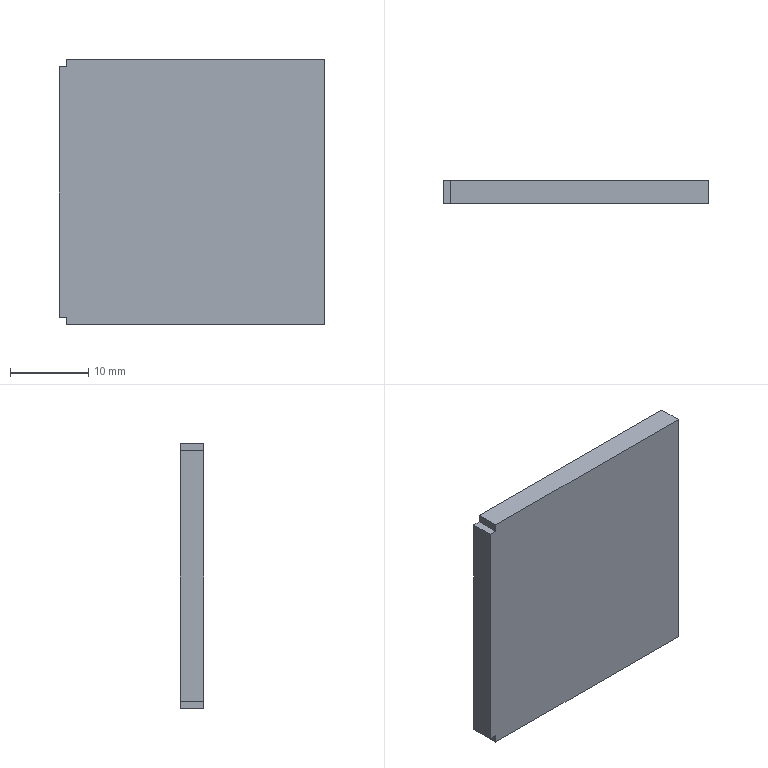Component | SolidWorks | CCQ-1.1-8WeldedPlate-4 | 1 solid | 10 faces | box 34 x 3 x 34 mm | volume 3462 mm3 | plane 10 | material 304
STEP:
#1=COLOUR_RGB('',0.7922,0.8196,0.9333);
#2=FILL_AREA_STYLE_COLOUR('',#1);
#3=FILL_AREA_STYLE('',(#2));
#4=SURFACE_STYLE_FILL_AREA(#3);
#5=SURFACE_SIDE_STYLE('',(#4));
#6=SURFACE_STYLE_USAGE(.BOTH.,#5);
#7=PRESENTATION_STYLE_ASSIGNMENT((#6));
#8=CARTESIAN_POINT('',(-25.866,-21.28,0.6299));
#9=VERTEX_POINT('',#8);
#10=CARTESIAN_POINT('',(-25.866,-21.398,0.6299));
#11=VERTEX_POINT('',#10);
#12=CARTESIAN_POINT('',(-25.866,-21.28,0.6299));
#13=DIRECTION('',(0.,-1.,0.));
#14=VECTOR('',#13,39.37);
#15=LINE('',#12,#14);
#16=EDGE_CURVE('',#9,#11,#15,.T.);
#17=ORIENTED_EDGE('',*,*,#16,.F.);
#18=CARTESIAN_POINT('',(-25.866,-21.28,-0.6299));
#19=VERTEX_POINT('',#18);
#20=CARTESIAN_POINT('',(-25.866,-21.28,-0.6693));
#21=DIRECTION('',(0.,-0.,-1.));
#22=VECTOR('',#21,39.37);
#23=LINE('',#20,#22);
#24=EDGE_CURVE('',#9,#19,#23,.T.);
#25=ORIENTED_EDGE('',*,*,#24,.T.);
#26=CARTESIAN_POINT('',(-25.866,-21.398,-0.6299));
#27=VERTEX_POINT('',#26);
#28=CARTESIAN_POINT('',(-25.866,-21.28,-0.6299));
#29=DIRECTION('',(-0.,1.,-0.));
#30=VECTOR('',#29,39.37);
#31=LINE('',#28,#30);
#32=EDGE_CURVE('',#27,#19,#31,.T.);
#33=ORIENTED_EDGE('',*,*,#32,.F.);
#34=CARTESIAN_POINT('',(-25.866,-21.398,-0.6693));
#35=DIRECTION('',(0.,-0.,-1.));
#36=VECTOR('',#35,39.37);
#37=LINE('',#34,#36);
#38=EDGE_CURVE('',#11,#27,#37,.T.);
#39=ORIENTED_EDGE('',*,*,#38,.F.);
#40=EDGE_LOOP('',(#17,#25,#33,#39));
#41=FACE_OUTER_BOUND('',#40,.T.);
#42=CARTESIAN_POINT('',(-25.866,-21.28,-0.6693));
#43=DIRECTION('',(-1.,-0.,-0.));
#44=DIRECTION('',(0.,-0.,-1.));
#45=AXIS2_PLACEMENT_3D('',#42,#43,#44);
#46=PLANE('',#45);
#47=ADVANCED_FACE('',(#41),#46,.T.);
#48=CARTESIAN_POINT('',(-25.827,-21.398,0.6693));
#49=VERTEX_POINT('',#48);
#50=CARTESIAN_POINT('',(-25.827,-21.28,0.6693));
#51=VERTEX_POINT('',#50);
#52=CARTESIAN_POINT('',(-25.827,-21.28,0.6693));
#53=DIRECTION('',(-0.,1.,-0.));
#54=VECTOR('',#53,39.37);
#55=LINE('',#52,#54);
#56=EDGE_CURVE('',#49,#51,#55,.T.);
#57=ORIENTED_EDGE('',*,*,#56,.F.);
#58=CARTESIAN_POINT('',(-24.528,-21.398,0.6693));
#59=VERTEX_POINT('',#58);
#60=CARTESIAN_POINT('',(-24.528,-21.398,0.6693));
#61=DIRECTION('',(-1.,-0.,0.));
#62=VECTOR('',#61,39.37);
#63=LINE('',#60,#62);
#64=EDGE_CURVE('',#59,#49,#63,.T.);
#65=ORIENTED_EDGE('',*,*,#64,.F.);
#66=CARTESIAN_POINT('',(-24.528,-21.28,0.6693));
#67=VERTEX_POINT('',#66);
#68=CARTESIAN_POINT('',(-24.528,-21.28,0.6693));
#69=DIRECTION('',(0.,-1.,0.));
#70=VECTOR('',#69,39.37);
#71=LINE('',#68,#70);
#72=EDGE_CURVE('',#67,#59,#71,.T.);
#73=ORIENTED_EDGE('',*,*,#72,.F.);
#74=CARTESIAN_POINT('',(-24.528,-21.28,0.6693));
#75=DIRECTION('',(-1.,-0.,0.));
#76=VECTOR('',#75,39.37);
#77=LINE('',#74,#76);
#78=EDGE_CURVE('',#67,#51,#77,.T.);
#79=ORIENTED_EDGE('',*,*,#78,.T.);
#80=EDGE_LOOP('',(#57,#65,#73,#79));
#81=FACE_OUTER_BOUND('',#80,.T.);
#82=CARTESIAN_POINT('',(-24.528,-21.28,0.6693));
#83=DIRECTION('',(0.,0.,1.));
#84=DIRECTION('',(-0.,1.,-0.));
#85=AXIS2_PLACEMENT_3D('',#82,#83,#84);
#86=PLANE('',#85);
#87=ADVANCED_FACE('',(#81),#86,.T.);
#88=CARTESIAN_POINT('',(-24.528,-21.398,-0.6693));
#89=VERTEX_POINT('',#88);
#90=CARTESIAN_POINT('',(-24.528,-21.398,-0.6693));
#91=DIRECTION('',(-0.,0.,1.));
#92=VECTOR('',#91,39.37);
#93=LINE('',#90,#92);
#94=EDGE_CURVE('',#89,#59,#93,.T.);
#95=ORIENTED_EDGE('',*,*,#94,.F.);
#96=CARTESIAN_POINT('',(-24.528,-21.28,-0.6693));
#97=VERTEX_POINT('',#96);
#98=CARTESIAN_POINT('',(-24.528,-21.28,-0.6693));
#99=DIRECTION('',(0.,-1.,0.));
#100=VECTOR('',#99,39.37);
#101=LINE('',#98,#100);
#102=EDGE_CURVE('',#97,#89,#101,.T.);
#103=ORIENTED_EDGE('',*,*,#102,.F.);
#104=CARTESIAN_POINT('',(-24.528,-21.28,-0.6693));
#105=DIRECTION('',(-0.,0.,1.));
#106=VECTOR('',#105,39.37);
#107=LINE('',#104,#106);
#108=EDGE_CURVE('',#97,#67,#107,.T.);
#109=ORIENTED_EDGE('',*,*,#108,.T.);
#110=ORIENTED_EDGE('',*,*,#72,.T.);
#111=EDGE_LOOP('',(#95,#103,#109,#110));
#112=FACE_OUTER_BOUND('',#111,.T.);
#113=CARTESIAN_POINT('',(-24.528,-21.28,-0.6693));
#114=DIRECTION('',(1.,0.,0.));
#115=DIRECTION('',(-0.,0.,1.));
#116=AXIS2_PLACEMENT_3D('',#113,#114,#115);
#117=PLANE('',#116);
#118=ADVANCED_FACE('',(#112),#117,.T.);
#119=CARTESIAN_POINT('',(-25.827,-21.28,-0.6693));
#120=VERTEX_POINT('',#119);
#121=CARTESIAN_POINT('',(-25.827,-21.398,-0.6693));
#122=VERTEX_POINT('',#121);
#123=CARTESIAN_POINT('',(-25.827,-21.28,-0.6693));
#124=DIRECTION('',(0.,-1.,0.));
#125=VECTOR('',#124,39.37);
#126=LINE('',#123,#125);
#127=EDGE_CURVE('',#120,#122,#126,.T.);
#128=ORIENTED_EDGE('',*,*,#127,.F.);
#129=CARTESIAN_POINT('',(-24.528,-21.28,-0.6693));
#130=DIRECTION('',(1.,0.,-0.));
#131=VECTOR('',#130,39.37);
#132=LINE('',#129,#131);
#133=EDGE_CURVE('',#120,#97,#132,.T.);
#134=ORIENTED_EDGE('',*,*,#133,.T.);
#135=ORIENTED_EDGE('',*,*,#102,.T.);
#136=CARTESIAN_POINT('',(-24.528,-21.398,-0.6693));
#137=DIRECTION('',(1.,0.,-0.));
#138=VECTOR('',#137,39.37);
#139=LINE('',#136,#138);
#140=EDGE_CURVE('',#122,#89,#139,.T.);
#141=ORIENTED_EDGE('',*,*,#140,.F.);
#142=EDGE_LOOP('',(#128,#134,#135,#141));
#143=FACE_OUTER_BOUND('',#142,.T.);
#144=CARTESIAN_POINT('',(-24.528,-21.28,-0.6693));
#145=DIRECTION('',(-0.,-0.,-1.));
#146=DIRECTION('',(0.,-1.,0.));
#147=AXIS2_PLACEMENT_3D('',#144,#145,#146);
#148=PLANE('',#147);
#149=ADVANCED_FACE('',(#143),#148,.T.);
#150=CARTESIAN_POINT('',(-25.827,-21.28,0.6299));
#151=VERTEX_POINT('',#150);
#152=CARTESIAN_POINT('',(-25.197,-21.28,0.6299));
#153=DIRECTION('',(1.,0.,-0.));
#154=VECTOR('',#153,39.37);
#155=LINE('',#152,#154);
#156=EDGE_CURVE('',#9,#151,#155,.T.);
#157=ORIENTED_EDGE('',*,*,#156,.T.);
#158=CARTESIAN_POINT('',(-25.827,-21.28,-0.));
#159=DIRECTION('',(0.,0.,1.));
#160=VECTOR('',#159,39.37);
#161=LINE('',#158,#160);
#162=EDGE_CURVE('',#151,#51,#161,.T.);
#163=ORIENTED_EDGE('',*,*,#162,.T.);
#164=ORIENTED_EDGE('',*,*,#78,.F.);
#165=ORIENTED_EDGE('',*,*,#108,.F.);
#166=ORIENTED_EDGE('',*,*,#133,.F.);
#167=CARTESIAN_POINT('',(-25.827,-21.28,-0.6299));
#168=VERTEX_POINT('',#167);
#169=CARTESIAN_POINT('',(-25.827,-21.28,-0.));
#170=DIRECTION('',(0.,0.,1.));
#171=VECTOR('',#170,39.37);
#172=LINE('',#169,#171);
#173=EDGE_CURVE('',#120,#168,#172,.T.);
#174=ORIENTED_EDGE('',*,*,#173,.T.);
#175=CARTESIAN_POINT('',(-25.197,-21.28,-0.6299));
#176=DIRECTION('',(-1.,-0.,0.));
#177=VECTOR('',#176,39.37);
#178=LINE('',#175,#177);
#179=EDGE_CURVE('',#168,#19,#178,.T.);
#180=ORIENTED_EDGE('',*,*,#179,.T.);
#181=ORIENTED_EDGE('',*,*,#24,.F.);
#182=EDGE_LOOP('',(#157,#163,#164,#165,#166,#174,#180,#181));
#183=FACE_OUTER_BOUND('',#182,.T.);
#184=CARTESIAN_POINT('',(-25.197,-21.28,-0.));
#185=DIRECTION('',(0.,-1.,0.));
#186=DIRECTION('',(-1.,-0.,0.));
#187=AXIS2_PLACEMENT_3D('',#184,#185,#186);
#188=PLANE('',#187);
#189=ADVANCED_FACE('',(#183),#188,.F.);
#190=CARTESIAN_POINT('',(-25.827,-21.398,0.6299));
#191=VERTEX_POINT('',#190);
#192=CARTESIAN_POINT('',(-25.827,-21.398,-0.));
#193=DIRECTION('',(0.,0.,1.));
#194=VECTOR('',#193,39.37);
#195=LINE('',#192,#194);
#196=EDGE_CURVE('',#191,#49,#195,.T.);
#197=ORIENTED_EDGE('',*,*,#196,.F.);
#198=CARTESIAN_POINT('',(-25.197,-21.398,0.6299));
#199=DIRECTION('',(1.,0.,-0.));
#200=VECTOR('',#199,39.37);
#201=LINE('',#198,#200);
#202=EDGE_CURVE('',#11,#191,#201,.T.);
#203=ORIENTED_EDGE('',*,*,#202,.F.);
#204=ORIENTED_EDGE('',*,*,#38,.T.);
#205=CARTESIAN_POINT('',(-25.827,-21.398,-0.6299));
#206=VERTEX_POINT('',#205);
#207=CARTESIAN_POINT('',(-25.197,-21.398,-0.6299));
#208=DIRECTION('',(-1.,-0.,0.));
#209=VECTOR('',#208,39.37);
#210=LINE('',#207,#209);
#211=EDGE_CURVE('',#206,#27,#210,.T.);
#212=ORIENTED_EDGE('',*,*,#211,.F.);
#213=CARTESIAN_POINT('',(-25.827,-21.398,-0.));
#214=DIRECTION('',(0.,0.,1.));
#215=VECTOR('',#214,39.37);
#216=LINE('',#213,#215);
#217=EDGE_CURVE('',#122,#206,#216,.T.);
#218=ORIENTED_EDGE('',*,*,#217,.F.);
#219=ORIENTED_EDGE('',*,*,#140,.T.);
#220=ORIENTED_EDGE('',*,*,#94,.T.);
#221=ORIENTED_EDGE('',*,*,#64,.T.);
#222=EDGE_LOOP('',(#197,#203,#204,#212,#218,#219,#220,#221));
#223=FACE_OUTER_BOUND('',#222,.T.);
#224=CARTESIAN_POINT('',(-25.197,-21.398,-0.));
#225=DIRECTION('',(0.,-1.,0.));
#226=DIRECTION('',(-1.,-0.,0.));
#227=AXIS2_PLACEMENT_3D('',#224,#225,#226);
#228=PLANE('',#227);
#229=ADVANCED_FACE('',(#223),#228,.T.);
#230=CARTESIAN_POINT('',(-25.827,-21.276,-0.6299));
#231=DIRECTION('',(0.,-1.,0.));
#232=VECTOR('',#231,39.37);
#233=LINE('',#230,#232);
#234=EDGE_CURVE('',#168,#206,#233,.T.);
#235=ORIENTED_EDGE('',*,*,#234,.T.);
#236=ORIENTED_EDGE('',*,*,#211,.T.);
#237=ORIENTED_EDGE('',*,*,#32,.T.);
#238=ORIENTED_EDGE('',*,*,#179,.F.);
#239=EDGE_LOOP('',(#235,#236,#237,#238));
#240=FACE_OUTER_BOUND('',#239,.T.);
#241=CARTESIAN_POINT('',(-25.848,-21.276,-0.6299));
#242=DIRECTION('',(0.,0.,1.));
#243=DIRECTION('',(-0.,1.,-0.));
#244=AXIS2_PLACEMENT_3D('',#241,#242,#243);
#245=PLANE('',#244);
#246=ADVANCED_FACE('',(#240),#245,.F.);
#247=ORIENTED_EDGE('',*,*,#127,.T.);
#248=ORIENTED_EDGE('',*,*,#217,.T.);
#249=ORIENTED_EDGE('',*,*,#234,.F.);
#250=ORIENTED_EDGE('',*,*,#173,.F.);
#251=EDGE_LOOP('',(#247,#248,#249,#250));
#252=FACE_OUTER_BOUND('',#251,.T.);
#253=CARTESIAN_POINT('',(-25.827,-21.276,-0.6516));
#254=DIRECTION('',(1.,0.,-0.));
#255=DIRECTION('',(0.,-1.,0.));
#256=AXIS2_PLACEMENT_3D('',#253,#254,#255);
#257=PLANE('',#256);
#258=ADVANCED_FACE('',(#252),#257,.F.);
#259=CARTESIAN_POINT('',(-25.827,-21.276,0.6299));
#260=DIRECTION('',(0.,-1.,0.));
#261=VECTOR('',#260,39.37);
#262=LINE('',#259,#261);
#263=EDGE_CURVE('',#151,#191,#262,.T.);
#264=ORIENTED_EDGE('',*,*,#263,.T.);
#265=ORIENTED_EDGE('',*,*,#196,.T.);
#266=ORIENTED_EDGE('',*,*,#56,.T.);
#267=ORIENTED_EDGE('',*,*,#162,.F.);
#268=EDGE_LOOP('',(#264,#265,#266,#267));
#269=FACE_OUTER_BOUND('',#268,.T.);
#270=CARTESIAN_POINT('',(-25.827,-21.276,0.6516));
#271=DIRECTION('',(1.,0.,-0.));
#272=DIRECTION('',(0.,-1.,0.));
#273=AXIS2_PLACEMENT_3D('',#270,#271,#272);
#274=PLANE('',#273);
#275=ADVANCED_FACE('',(#269),#274,.F.);
#276=ORIENTED_EDGE('',*,*,#16,.T.);
#277=ORIENTED_EDGE('',*,*,#202,.T.);
#278=ORIENTED_EDGE('',*,*,#263,.F.);
#279=ORIENTED_EDGE('',*,*,#156,.F.);
#280=EDGE_LOOP('',(#276,#277,#278,#279));
#281=FACE_OUTER_BOUND('',#280,.T.);
#282=CARTESIAN_POINT('',(-25.848,-21.276,0.6299));
#283=DIRECTION('',(-0.,-0.,-1.));
#284=DIRECTION('',(0.,-1.,0.));
#285=AXIS2_PLACEMENT_3D('',#282,#283,#284);
#286=PLANE('',#285);
#287=ADVANCED_FACE('',(#281),#286,.F.);
#288=CLOSED_SHELL('',(#47,#87,#118,#149,#189,#229,#246,#258,#275,#287));
#289=MANIFOLD_SOLID_BREP('',#288);
#290=STYLED_ITEM('',(#7),#289);
#291=(LENGTH_UNIT()NAMED_UNIT(*)SI_UNIT($,.METRE.));
#292=LENGTH_MEASURE_WITH_UNIT(LENGTH_MEASURE(0.0254),#291);
#293=DIMENSIONAL_EXPONENTS(1.,0.,0.,0.,0.,0.,0.);
#294=(CONVERSION_BASED_UNIT('',#292)LENGTH_UNIT()NAMED_UNIT(#293));
#295=UNCERTAINTY_MEASURE_WITH_UNIT(LENGTH_MEASURE(0.00001),#294,'','');
#296=(NAMED_UNIT(*)PLANE_ANGLE_UNIT()SI_UNIT($,.RADIAN.));
#297=(NAMED_UNIT(*)SI_UNIT($,.STERADIAN.)SOLID_ANGLE_UNIT());
#298=(GEOMETRIC_REPRESENTATION_CONTEXT(3)GLOBAL_UNCERTAINTY_ASSIGNED_CONTEXT((#295))GLOBAL_UNIT_ASSIGNED_CONTEXT((#294,#296,#297))REPRESENTATION_CONTEXT('',''));
#299=MECHANICAL_DESIGN_GEOMETRIC_PRESENTATION_REPRESENTATION('',(#290),#298);
#300=PRESENTATION_LAYER_ASSIGNMENT('','',(#290));
#301=CARTESIAN_POINT('',(0.,0.,0.));
#302=DIRECTION('',(0.,0.,1.));
#303=DIRECTION('',(1.,0.,0.));
#304=AXIS2_PLACEMENT_3D('',#301,#302,#303);
#305=(LENGTH_UNIT()NAMED_UNIT(*)SI_UNIT($,.METRE.));
#306=LENGTH_MEASURE_WITH_UNIT(LENGTH_MEASURE(0.0254),#305);
#307=DIMENSIONAL_EXPONENTS(1.,0.,0.,0.,0.,0.,0.);
#308=(CONVERSION_BASED_UNIT('',#306)LENGTH_UNIT()NAMED_UNIT(#307));
#309=UNCERTAINTY_MEASURE_WITH_UNIT(LENGTH_MEASURE(0.00001),#308,'','');
#310=(NAMED_UNIT(*)PLANE_ANGLE_UNIT()SI_UNIT($,.RADIAN.));
#311=(NAMED_UNIT(*)SI_UNIT($,.STERADIAN.)SOLID_ANGLE_UNIT());
#312=(GEOMETRIC_REPRESENTATION_CONTEXT(3)GLOBAL_UNCERTAINTY_ASSIGNED_CONTEXT((#309))GLOBAL_UNIT_ASSIGNED_CONTEXT((#308,#310,#311))REPRESENTATION_CONTEXT('',''));
#313=ADVANCED_BREP_SHAPE_REPRESENTATION('',(#289,#304),#312);